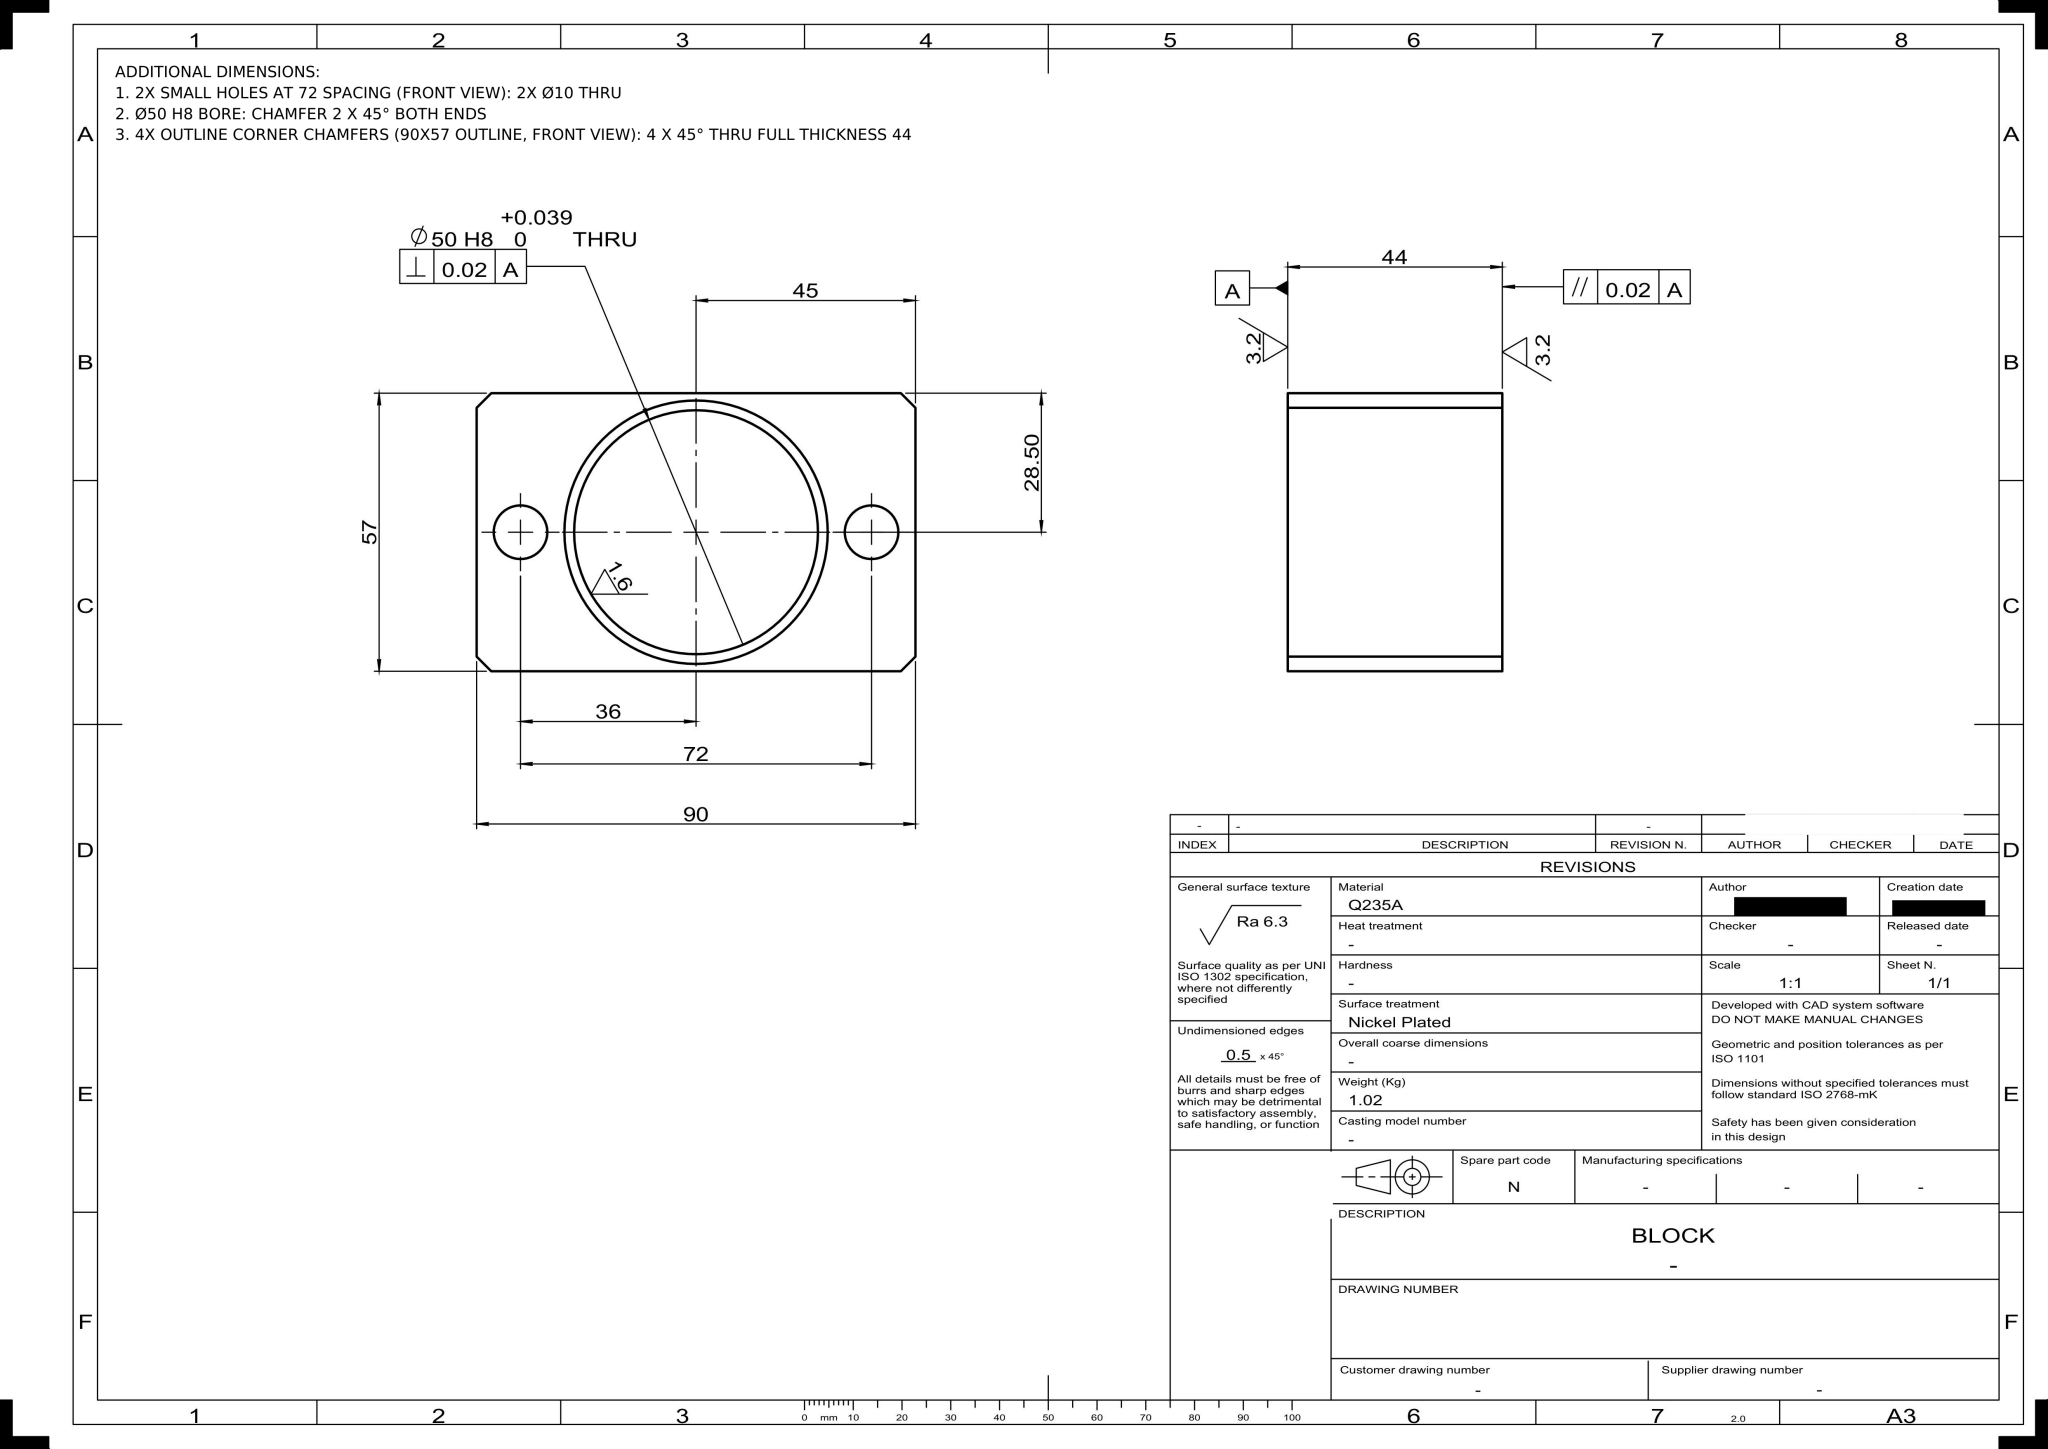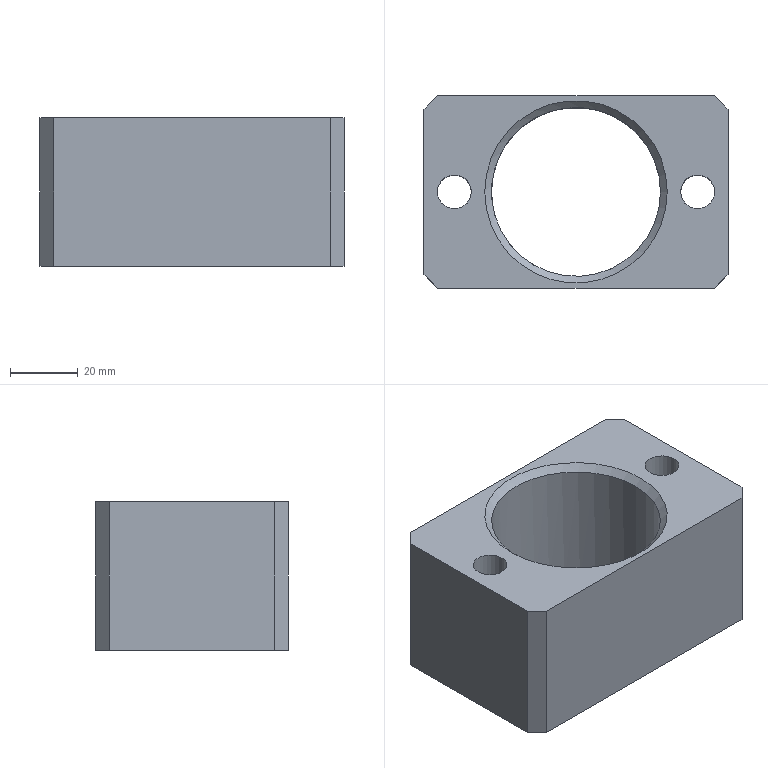Part | NX | mm | 1 solid | 15 faces | box 90 x 57 x 44 mm | volume 130362 mm3 | plane 10 | cylinder 3 | cone 2 | commonest cylinder face diameters 10 x2 50 x1
STEP:
#1=CARTESIAN_POINT('',(0.,0.,0.));
#2=DIRECTION('',(0.,0.,1.));
#3=DIRECTION('',(1.,0.,0.));
#4=AXIS2_PLACEMENT_3D('',#1,#2,#3);
#5=(LENGTH_UNIT()NAMED_UNIT(*)SI_UNIT(.MILLI.,.METRE.));
#6=UNCERTAINTY_MEASURE_WITH_UNIT(LENGTH_MEASURE(0.00002),#5,'','');
#7=(NAMED_UNIT(*)PLANE_ANGLE_UNIT()SI_UNIT($,.RADIAN.));
#8=PLANE_ANGLE_MEASURE_WITH_UNIT(PLANE_ANGLE_MEASURE(0.01745),#7);
#9=DIMENSIONAL_EXPONENTS(0.,0.,0.,0.,0.,0.,0.);
#10=(CONVERSION_BASED_UNIT('',#8)NAMED_UNIT(#9)PLANE_ANGLE_UNIT());
#11=(NAMED_UNIT(*)SI_UNIT($,.STERADIAN.)SOLID_ANGLE_UNIT());
#12=(GEOMETRIC_REPRESENTATION_CONTEXT(3)GLOBAL_UNCERTAINTY_ASSIGNED_CONTEXT((#6))GLOBAL_UNIT_ASSIGNED_CONTEXT((#5,#10,#11))REPRESENTATION_CONTEXT('',''));
#13=SHAPE_REPRESENTATION('',(#4),#12);
#14=CARTESIAN_POINT('',(-45.,24.5,44.));
#15=VERTEX_POINT('',#14);
#16=CARTESIAN_POINT('',(-45.,-24.5,44.));
#17=VERTEX_POINT('',#16);
#18=CARTESIAN_POINT('',(-45.,28.5,44.));
#19=DIRECTION('',(0.,-1.,0.));
#20=VECTOR('',#19,1.);
#21=LINE('',#18,#20);
#22=EDGE_CURVE('',#15,#17,#21,.T.);
#23=ORIENTED_EDGE('',*,*,#22,.F.);
#24=CARTESIAN_POINT('',(-45.,24.5,0.));
#25=VERTEX_POINT('',#24);
#26=CARTESIAN_POINT('',(-45.,24.5,44.));
#27=DIRECTION('',(0.,0.,-1.));
#28=VECTOR('',#27,1.);
#29=LINE('',#26,#28);
#30=EDGE_CURVE('',#15,#25,#29,.T.);
#31=ORIENTED_EDGE('',*,*,#30,.T.);
#32=CARTESIAN_POINT('',(-45.,-24.5,0.));
#33=VERTEX_POINT('',#32);
#34=CARTESIAN_POINT('',(-45.,28.5,0.));
#35=DIRECTION('',(0.,-1.,0.));
#36=VECTOR('',#35,1.);
#37=LINE('',#34,#36);
#38=EDGE_CURVE('',#25,#33,#37,.T.);
#39=ORIENTED_EDGE('',*,*,#38,.T.);
#40=CARTESIAN_POINT('',(-45.,-24.5,44.));
#41=DIRECTION('',(0.,0.,1.));
#42=VECTOR('',#41,1.);
#43=LINE('',#40,#42);
#44=EDGE_CURVE('',#33,#17,#43,.T.);
#45=ORIENTED_EDGE('',*,*,#44,.T.);
#46=EDGE_LOOP('',(#23,#31,#39,#45));
#47=FACE_OUTER_BOUND('',#46,.T.);
#48=CARTESIAN_POINT('',(-45.,28.5,44.));
#49=DIRECTION('',(1.,0.,0.));
#50=DIRECTION('',(-0.,1.,0.));
#51=AXIS2_PLACEMENT_3D('',#48,#49,#50);
#52=PLANE('',#51);
#53=ADVANCED_FACE('',(#47),#52,.F.);
#54=CARTESIAN_POINT('',(-41.,-28.5,0.));
#55=VERTEX_POINT('',#54);
#56=CARTESIAN_POINT('',(41.,-28.5,0.));
#57=VERTEX_POINT('',#56);
#58=CARTESIAN_POINT('',(-45.,-28.5,0.));
#59=DIRECTION('',(1.,0.,0.));
#60=VECTOR('',#59,1.);
#61=LINE('',#58,#60);
#62=EDGE_CURVE('',#55,#57,#61,.T.);
#63=ORIENTED_EDGE('',*,*,#62,.T.);
#64=CARTESIAN_POINT('',(41.,-28.5,44.));
#65=VERTEX_POINT('',#64);
#66=CARTESIAN_POINT('',(41.,-28.5,44.));
#67=DIRECTION('',(0.,0.,1.));
#68=VECTOR('',#67,1.);
#69=LINE('',#66,#68);
#70=EDGE_CURVE('',#57,#65,#69,.T.);
#71=ORIENTED_EDGE('',*,*,#70,.T.);
#72=CARTESIAN_POINT('',(-41.,-28.5,44.));
#73=VERTEX_POINT('',#72);
#74=CARTESIAN_POINT('',(-45.,-28.5,44.));
#75=DIRECTION('',(1.,0.,0.));
#76=VECTOR('',#75,1.);
#77=LINE('',#74,#76);
#78=EDGE_CURVE('',#73,#65,#77,.T.);
#79=ORIENTED_EDGE('',*,*,#78,.F.);
#80=CARTESIAN_POINT('',(-41.,-28.5,44.));
#81=DIRECTION('',(0.,0.,-1.));
#82=VECTOR('',#81,1.);
#83=LINE('',#80,#82);
#84=EDGE_CURVE('',#73,#55,#83,.T.);
#85=ORIENTED_EDGE('',*,*,#84,.T.);
#86=EDGE_LOOP('',(#63,#71,#79,#85));
#87=FACE_OUTER_BOUND('',#86,.T.);
#88=CARTESIAN_POINT('',(-45.,-28.5,44.));
#89=DIRECTION('',(0.,1.,0.));
#90=DIRECTION('',(0.,0.,1.));
#91=AXIS2_PLACEMENT_3D('',#88,#89,#90);
#92=PLANE('',#91);
#93=ADVANCED_FACE('',(#87),#92,.F.);
#94=CARTESIAN_POINT('',(45.,-24.5,44.));
#95=VERTEX_POINT('',#94);
#96=CARTESIAN_POINT('',(45.,24.5,44.));
#97=VERTEX_POINT('',#96);
#98=CARTESIAN_POINT('',(45.,-28.5,44.));
#99=DIRECTION('',(-0.,1.,0.));
#100=VECTOR('',#99,1.);
#101=LINE('',#98,#100);
#102=EDGE_CURVE('',#95,#97,#101,.T.);
#103=ORIENTED_EDGE('',*,*,#102,.F.);
#104=CARTESIAN_POINT('',(45.,-24.5,0.));
#105=VERTEX_POINT('',#104);
#106=CARTESIAN_POINT('',(45.,-24.5,44.));
#107=DIRECTION('',(0.,0.,-1.));
#108=VECTOR('',#107,1.);
#109=LINE('',#106,#108);
#110=EDGE_CURVE('',#95,#105,#109,.T.);
#111=ORIENTED_EDGE('',*,*,#110,.T.);
#112=CARTESIAN_POINT('',(45.,24.5,0.));
#113=VERTEX_POINT('',#112);
#114=CARTESIAN_POINT('',(45.,-28.5,0.));
#115=DIRECTION('',(-0.,1.,0.));
#116=VECTOR('',#115,1.);
#117=LINE('',#114,#116);
#118=EDGE_CURVE('',#105,#113,#117,.T.);
#119=ORIENTED_EDGE('',*,*,#118,.T.);
#120=CARTESIAN_POINT('',(45.,24.5,44.));
#121=DIRECTION('',(0.,0.,1.));
#122=VECTOR('',#121,1.);
#123=LINE('',#120,#122);
#124=EDGE_CURVE('',#113,#97,#123,.T.);
#125=ORIENTED_EDGE('',*,*,#124,.T.);
#126=EDGE_LOOP('',(#103,#111,#119,#125));
#127=FACE_OUTER_BOUND('',#126,.T.);
#128=CARTESIAN_POINT('',(45.,-28.5,44.));
#129=DIRECTION('',(-1.,-0.,0.));
#130=DIRECTION('',(0.,-1.,0.));
#131=AXIS2_PLACEMENT_3D('',#128,#129,#130);
#132=PLANE('',#131);
#133=ADVANCED_FACE('',(#127),#132,.F.);
#134=CARTESIAN_POINT('',(41.,28.5,44.));
#135=VERTEX_POINT('',#134);
#136=CARTESIAN_POINT('',(-41.,28.5,44.));
#137=VERTEX_POINT('',#136);
#138=CARTESIAN_POINT('',(45.,28.5,44.));
#139=DIRECTION('',(-1.,0.,0.));
#140=VECTOR('',#139,1.);
#141=LINE('',#138,#140);
#142=EDGE_CURVE('',#135,#137,#141,.T.);
#143=ORIENTED_EDGE('',*,*,#142,.F.);
#144=CARTESIAN_POINT('',(41.,28.5,0.));
#145=VERTEX_POINT('',#144);
#146=CARTESIAN_POINT('',(41.,28.5,44.));
#147=DIRECTION('',(0.,0.,-1.));
#148=VECTOR('',#147,1.);
#149=LINE('',#146,#148);
#150=EDGE_CURVE('',#135,#145,#149,.T.);
#151=ORIENTED_EDGE('',*,*,#150,.T.);
#152=CARTESIAN_POINT('',(-41.,28.5,0.));
#153=VERTEX_POINT('',#152);
#154=CARTESIAN_POINT('',(45.,28.5,0.));
#155=DIRECTION('',(-1.,0.,0.));
#156=VECTOR('',#155,1.);
#157=LINE('',#154,#156);
#158=EDGE_CURVE('',#145,#153,#157,.T.);
#159=ORIENTED_EDGE('',*,*,#158,.T.);
#160=CARTESIAN_POINT('',(-41.,28.5,44.));
#161=DIRECTION('',(0.,0.,1.));
#162=VECTOR('',#161,1.);
#163=LINE('',#160,#162);
#164=EDGE_CURVE('',#153,#137,#163,.T.);
#165=ORIENTED_EDGE('',*,*,#164,.T.);
#166=EDGE_LOOP('',(#143,#151,#159,#165));
#167=FACE_OUTER_BOUND('',#166,.T.);
#168=CARTESIAN_POINT('',(45.,28.5,44.));
#169=DIRECTION('',(0.,-1.,0.));
#170=DIRECTION('',(0.,0.,-1.));
#171=AXIS2_PLACEMENT_3D('',#168,#169,#170);
#172=PLANE('',#171);
#173=ADVANCED_FACE('',(#167),#172,.F.);
#174=CARTESIAN_POINT('',(31.,0.,44.));
#175=VERTEX_POINT('',#174);
#176=CARTESIAN_POINT('',(36.,0.,44.));
#177=DIRECTION('',(0.,0.,-1.));
#178=DIRECTION('',(-1.,0.,0.));
#179=AXIS2_PLACEMENT_3D('',#176,#177,#178);
#180=CIRCLE('',#179,5.);
#181=EDGE_CURVE('',#175,#175,#180,.T.);
#182=ORIENTED_EDGE('',*,*,#181,.T.);
#183=EDGE_LOOP('',(#182));
#184=FACE_BOUND('',#183,.T.);
#185=CARTESIAN_POINT('',(-41.,0.,44.));
#186=VERTEX_POINT('',#185);
#187=CARTESIAN_POINT('',(-36.,0.,44.));
#188=DIRECTION('',(0.,0.,-1.));
#189=DIRECTION('',(-1.,0.,0.));
#190=AXIS2_PLACEMENT_3D('',#187,#188,#189);
#191=CIRCLE('',#190,5.);
#192=EDGE_CURVE('',#186,#186,#191,.T.);
#193=ORIENTED_EDGE('',*,*,#192,.T.);
#194=EDGE_LOOP('',(#193));
#195=FACE_BOUND('',#194,.T.);
#196=CARTESIAN_POINT('',(27.,0.,44.));
#197=VERTEX_POINT('',#196);
#198=CARTESIAN_POINT('',(0.,0.,44.));
#199=DIRECTION('',(0.,0.,1.));
#200=DIRECTION('',(1.,0.,0.));
#201=AXIS2_PLACEMENT_3D('',#198,#199,#200);
#202=CIRCLE('',#201,27.);
#203=EDGE_CURVE('',#197,#197,#202,.T.);
#204=ORIENTED_EDGE('',*,*,#203,.F.);
#205=EDGE_LOOP('',(#204));
#206=FACE_BOUND('',#205,.T.);
#207=ORIENTED_EDGE('',*,*,#78,.T.);
#208=CARTESIAN_POINT('',(34.75,-34.75,44.));
#209=DIRECTION('',(0.7071,0.7071,0.));
#210=VECTOR('',#209,1.);
#211=LINE('',#208,#210);
#212=EDGE_CURVE('',#65,#95,#211,.T.);
#213=ORIENTED_EDGE('',*,*,#212,.T.);
#214=ORIENTED_EDGE('',*,*,#102,.T.);
#215=CARTESIAN_POINT('',(34.75,34.75,44.));
#216=DIRECTION('',(-0.7071,0.7071,0.));
#217=VECTOR('',#216,1.);
#218=LINE('',#215,#217);
#219=EDGE_CURVE('',#97,#135,#218,.T.);
#220=ORIENTED_EDGE('',*,*,#219,.T.);
#221=ORIENTED_EDGE('',*,*,#142,.T.);
#222=CARTESIAN_POINT('',(-34.75,34.75,44.));
#223=DIRECTION('',(-0.7071,-0.7071,0.));
#224=VECTOR('',#223,1.);
#225=LINE('',#222,#224);
#226=EDGE_CURVE('',#137,#15,#225,.T.);
#227=ORIENTED_EDGE('',*,*,#226,.T.);
#228=ORIENTED_EDGE('',*,*,#22,.T.);
#229=CARTESIAN_POINT('',(-34.75,-34.75,44.));
#230=DIRECTION('',(0.7071,-0.7071,0.));
#231=VECTOR('',#230,1.);
#232=LINE('',#229,#231);
#233=EDGE_CURVE('',#17,#73,#232,.T.);
#234=ORIENTED_EDGE('',*,*,#233,.T.);
#235=EDGE_LOOP('',(#207,#213,#214,#220,#221,#227,#228,#234));
#236=FACE_BOUND('',#235,.T.);
#237=CARTESIAN_POINT('',(0.,0.,44.));
#238=DIRECTION('',(0.,0.,1.));
#239=DIRECTION('',(1.,0.,0.));
#240=AXIS2_PLACEMENT_3D('',#237,#238,#239);
#241=PLANE('',#240);
#242=ADVANCED_FACE('',(#184,#195,#206,#236),#241,.T.);
#243=CARTESIAN_POINT('',(41.,0.,0.));
#244=VERTEX_POINT('',#243);
#245=CARTESIAN_POINT('',(36.,0.,0.));
#246=DIRECTION('',(0.,0.,1.));
#247=DIRECTION('',(1.,0.,0.));
#248=AXIS2_PLACEMENT_3D('',#245,#246,#247);
#249=CIRCLE('',#248,5.);
#250=EDGE_CURVE('',#244,#244,#249,.T.);
#251=ORIENTED_EDGE('',*,*,#250,.T.);
#252=EDGE_LOOP('',(#251));
#253=FACE_BOUND('',#252,.T.);
#254=CARTESIAN_POINT('',(-31.,0.,0.));
#255=VERTEX_POINT('',#254);
#256=CARTESIAN_POINT('',(-36.,0.,0.));
#257=DIRECTION('',(0.,0.,1.));
#258=DIRECTION('',(1.,0.,0.));
#259=AXIS2_PLACEMENT_3D('',#256,#257,#258);
#260=CIRCLE('',#259,5.);
#261=EDGE_CURVE('',#255,#255,#260,.T.);
#262=ORIENTED_EDGE('',*,*,#261,.T.);
#263=EDGE_LOOP('',(#262));
#264=FACE_BOUND('',#263,.T.);
#265=CARTESIAN_POINT('',(27.,0.,0.));
#266=VERTEX_POINT('',#265);
#267=CARTESIAN_POINT('',(0.,0.,0.));
#268=DIRECTION('',(0.,0.,1.));
#269=DIRECTION('',(1.,0.,0.));
#270=AXIS2_PLACEMENT_3D('',#267,#268,#269);
#271=CIRCLE('',#270,27.);
#272=EDGE_CURVE('',#266,#266,#271,.T.);
#273=ORIENTED_EDGE('',*,*,#272,.T.);
#274=EDGE_LOOP('',(#273));
#275=FACE_BOUND('',#274,.T.);
#276=ORIENTED_EDGE('',*,*,#118,.F.);
#277=CARTESIAN_POINT('',(45.,-24.5,0.));
#278=DIRECTION('',(-0.7071,-0.7071,0.));
#279=VECTOR('',#278,1.);
#280=LINE('',#277,#279);
#281=EDGE_CURVE('',#105,#57,#280,.T.);
#282=ORIENTED_EDGE('',*,*,#281,.T.);
#283=ORIENTED_EDGE('',*,*,#62,.F.);
#284=CARTESIAN_POINT('',(-41.,-28.5,0.));
#285=DIRECTION('',(-0.7071,0.7071,0.));
#286=VECTOR('',#285,1.);
#287=LINE('',#284,#286);
#288=EDGE_CURVE('',#55,#33,#287,.T.);
#289=ORIENTED_EDGE('',*,*,#288,.T.);
#290=ORIENTED_EDGE('',*,*,#38,.F.);
#291=CARTESIAN_POINT('',(-45.,24.5,0.));
#292=DIRECTION('',(0.7071,0.7071,0.));
#293=VECTOR('',#292,1.);
#294=LINE('',#291,#293);
#295=EDGE_CURVE('',#25,#153,#294,.T.);
#296=ORIENTED_EDGE('',*,*,#295,.T.);
#297=ORIENTED_EDGE('',*,*,#158,.F.);
#298=CARTESIAN_POINT('',(41.,28.5,0.));
#299=DIRECTION('',(0.7071,-0.7071,0.));
#300=VECTOR('',#299,1.);
#301=LINE('',#298,#300);
#302=EDGE_CURVE('',#145,#113,#301,.T.);
#303=ORIENTED_EDGE('',*,*,#302,.T.);
#304=EDGE_LOOP('',(#276,#282,#283,#289,#290,#296,#297,#303));
#305=FACE_BOUND('',#304,.T.);
#306=CARTESIAN_POINT('',(0.,0.,0.));
#307=DIRECTION('',(0.,0.,1.));
#308=DIRECTION('',(1.,0.,0.));
#309=AXIS2_PLACEMENT_3D('',#306,#307,#308);
#310=PLANE('',#309);
#311=ADVANCED_FACE('',(#253,#264,#275,#305),#310,.F.);
#312=CARTESIAN_POINT('',(25.,0.,42.));
#313=VERTEX_POINT('',#312);
#314=CARTESIAN_POINT('',(0.,0.,42.));
#315=DIRECTION('',(0.,0.,1.));
#316=DIRECTION('',(1.,0.,0.));
#317=AXIS2_PLACEMENT_3D('',#314,#315,#316);
#318=CIRCLE('',#317,25.);
#319=EDGE_CURVE('',#313,#313,#318,.T.);
#320=ORIENTED_EDGE('',*,*,#319,.T.);
#321=EDGE_LOOP('',(#320));
#322=FACE_BOUND('',#321,.T.);
#323=CARTESIAN_POINT('',(-25.,0.,2.));
#324=VERTEX_POINT('',#323);
#325=CARTESIAN_POINT('',(0.,0.,2.));
#326=DIRECTION('',(0.,0.,-1.));
#327=DIRECTION('',(-1.,0.,0.));
#328=AXIS2_PLACEMENT_3D('',#325,#326,#327);
#329=CIRCLE('',#328,25.);
#330=EDGE_CURVE('',#324,#324,#329,.T.);
#331=ORIENTED_EDGE('',*,*,#330,.T.);
#332=EDGE_LOOP('',(#331));
#333=FACE_BOUND('',#332,.T.);
#334=CARTESIAN_POINT('',(0.,0.,0.));
#335=DIRECTION('',(0.,0.,1.));
#336=DIRECTION('',(1.,0.,0.));
#337=AXIS2_PLACEMENT_3D('',#334,#335,#336);
#338=CYLINDRICAL_SURFACE('',#337,25.);
#339=ADVANCED_FACE('',(#322,#333),#338,.F.);
#340=ORIENTED_EDGE('',*,*,#330,.F.);
#341=EDGE_LOOP('',(#340));
#342=FACE_BOUND('',#341,.T.);
#343=ORIENTED_EDGE('',*,*,#272,.F.);
#344=EDGE_LOOP('',(#343));
#345=FACE_BOUND('',#344,.T.);
#346=CARTESIAN_POINT('',(0.,0.,27.));
#347=DIRECTION('',(0.,0.,-1.));
#348=DIRECTION('',(-1.,0.,-0.));
#349=AXIS2_PLACEMENT_3D('',#346,#347,#348);
#350=CONICAL_SURFACE('',#349,0.,45.);
#351=ADVANCED_FACE('',(#342,#345),#350,.F.);
#352=ORIENTED_EDGE('',*,*,#203,.T.);
#353=EDGE_LOOP('',(#352));
#354=FACE_BOUND('',#353,.T.);
#355=ORIENTED_EDGE('',*,*,#319,.F.);
#356=EDGE_LOOP('',(#355));
#357=FACE_BOUND('',#356,.T.);
#358=CARTESIAN_POINT('',(0.,0.,17.));
#359=DIRECTION('',(0.,0.,1.));
#360=DIRECTION('',(1.,0.,-0.));
#361=AXIS2_PLACEMENT_3D('',#358,#359,#360);
#362=CONICAL_SURFACE('',#361,0.,45.);
#363=ADVANCED_FACE('',(#354,#357),#362,.F.);
#364=ORIENTED_EDGE('',*,*,#192,.F.);
#365=EDGE_LOOP('',(#364));
#366=FACE_BOUND('',#365,.T.);
#367=ORIENTED_EDGE('',*,*,#261,.F.);
#368=EDGE_LOOP('',(#367));
#369=FACE_BOUND('',#368,.T.);
#370=CARTESIAN_POINT('',(-36.,0.,44.));
#371=DIRECTION('',(0.,0.,-1.));
#372=DIRECTION('',(-1.,0.,0.));
#373=AXIS2_PLACEMENT_3D('',#370,#371,#372);
#374=CYLINDRICAL_SURFACE('',#373,5.);
#375=ADVANCED_FACE('',(#366,#369),#374,.F.);
#376=ORIENTED_EDGE('',*,*,#181,.F.);
#377=EDGE_LOOP('',(#376));
#378=FACE_BOUND('',#377,.T.);
#379=ORIENTED_EDGE('',*,*,#250,.F.);
#380=EDGE_LOOP('',(#379));
#381=FACE_BOUND('',#380,.T.);
#382=CARTESIAN_POINT('',(36.,0.,44.));
#383=DIRECTION('',(0.,0.,-1.));
#384=DIRECTION('',(-1.,0.,0.));
#385=AXIS2_PLACEMENT_3D('',#382,#383,#384);
#386=CYLINDRICAL_SURFACE('',#385,5.);
#387=ADVANCED_FACE('',(#378,#381),#386,.F.);
#388=ORIENTED_EDGE('',*,*,#212,.F.);
#389=ORIENTED_EDGE('',*,*,#70,.F.);
#390=ORIENTED_EDGE('',*,*,#281,.F.);
#391=ORIENTED_EDGE('',*,*,#110,.F.);
#392=EDGE_LOOP('',(#388,#389,#390,#391));
#393=FACE_OUTER_BOUND('',#392,.T.);
#394=CARTESIAN_POINT('',(45.,-24.5,44.));
#395=DIRECTION('',(-0.7071,0.7071,0.));
#396=DIRECTION('',(0.,0.,-1.));
#397=AXIS2_PLACEMENT_3D('',#394,#395,#396);
#398=PLANE('',#397);
#399=ADVANCED_FACE('',(#393),#398,.F.);
#400=ORIENTED_EDGE('',*,*,#219,.F.);
#401=ORIENTED_EDGE('',*,*,#124,.F.);
#402=ORIENTED_EDGE('',*,*,#302,.F.);
#403=ORIENTED_EDGE('',*,*,#150,.F.);
#404=EDGE_LOOP('',(#400,#401,#402,#403));
#405=FACE_OUTER_BOUND('',#404,.T.);
#406=CARTESIAN_POINT('',(41.,28.5,44.));
#407=DIRECTION('',(-0.7071,-0.7071,0.));
#408=DIRECTION('',(0.,0.,-1.));
#409=AXIS2_PLACEMENT_3D('',#406,#407,#408);
#410=PLANE('',#409);
#411=ADVANCED_FACE('',(#405),#410,.F.);
#412=ORIENTED_EDGE('',*,*,#226,.F.);
#413=ORIENTED_EDGE('',*,*,#164,.F.);
#414=ORIENTED_EDGE('',*,*,#295,.F.);
#415=ORIENTED_EDGE('',*,*,#30,.F.);
#416=EDGE_LOOP('',(#412,#413,#414,#415));
#417=FACE_OUTER_BOUND('',#416,.T.);
#418=CARTESIAN_POINT('',(-45.,24.5,44.));
#419=DIRECTION('',(0.7071,-0.7071,0.));
#420=DIRECTION('',(0.,0.,-1.));
#421=AXIS2_PLACEMENT_3D('',#418,#419,#420);
#422=PLANE('',#421);
#423=ADVANCED_FACE('',(#417),#422,.F.);
#424=ORIENTED_EDGE('',*,*,#233,.F.);
#425=ORIENTED_EDGE('',*,*,#44,.F.);
#426=ORIENTED_EDGE('',*,*,#288,.F.);
#427=ORIENTED_EDGE('',*,*,#84,.F.);
#428=EDGE_LOOP('',(#424,#425,#426,#427));
#429=FACE_OUTER_BOUND('',#428,.T.);
#430=CARTESIAN_POINT('',(-41.,-28.5,44.));
#431=DIRECTION('',(0.7071,0.7071,0.));
#432=DIRECTION('',(0.,0.,-1.));
#433=AXIS2_PLACEMENT_3D('',#430,#431,#432);
#434=PLANE('',#433);
#435=ADVANCED_FACE('',(#429),#434,.F.);
#436=CLOSED_SHELL('',(#53,#93,#133,#173,#242,#311,#339,#351,#363,#375,#387,#399,#411,#423,#435));
#437=MANIFOLD_SOLID_BREP('',#436);
#438=ADVANCED_BREP_SHAPE_REPRESENTATION('',(#437),#12);
#439=SHAPE_REPRESENTATION_RELATIONSHIP('','',#13,#438);
#440=PRESENTATION_LAYER_ASSIGNMENT('','',(#437));
#441=COLOUR_RGB('',0.4,0.8,1.);
#442=FILL_AREA_STYLE_COLOUR('',#441);
#443=FILL_AREA_STYLE('',(#442));
#444=SURFACE_STYLE_FILL_AREA(#443);
#445=SURFACE_SIDE_STYLE('',(#444));
#446=SURFACE_STYLE_USAGE(.BOTH.,#445);
#447=PRESENTATION_STYLE_ASSIGNMENT((#446));
#448=STYLED_ITEM('',(#447),#437);
#449=MECHANICAL_DESIGN_GEOMETRIC_PRESENTATION_REPRESENTATION('',(#448),#12);